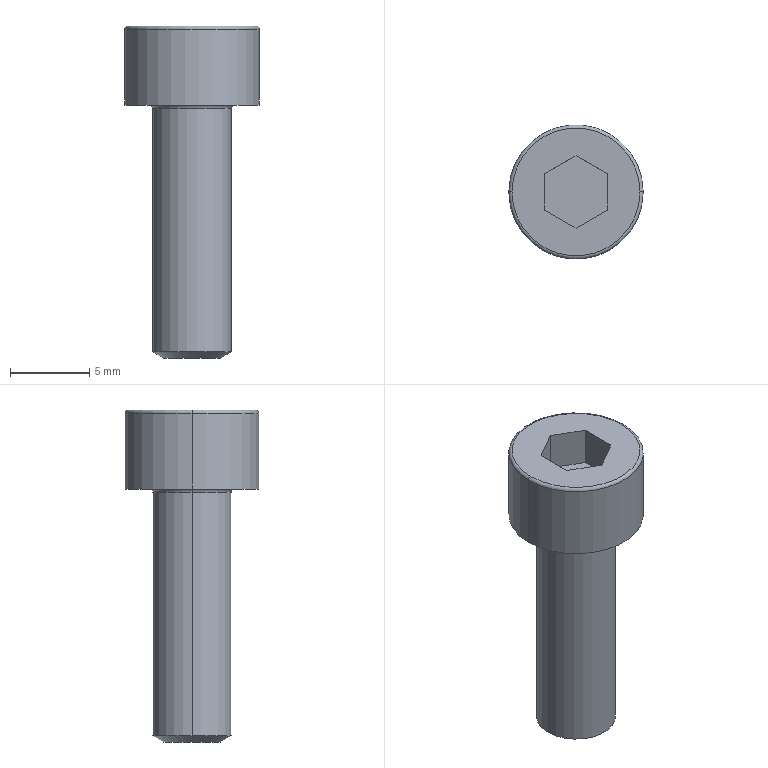Component | NX | HEX_SOCKET_CAP_SCREW_M5X16 | 1 solid | 20 faces | volume 562 mm3 | plane 10 | torus 4 | cylinder 4 | cone 2 | commonest cylinder face diameters 8.5 x2 5 x2